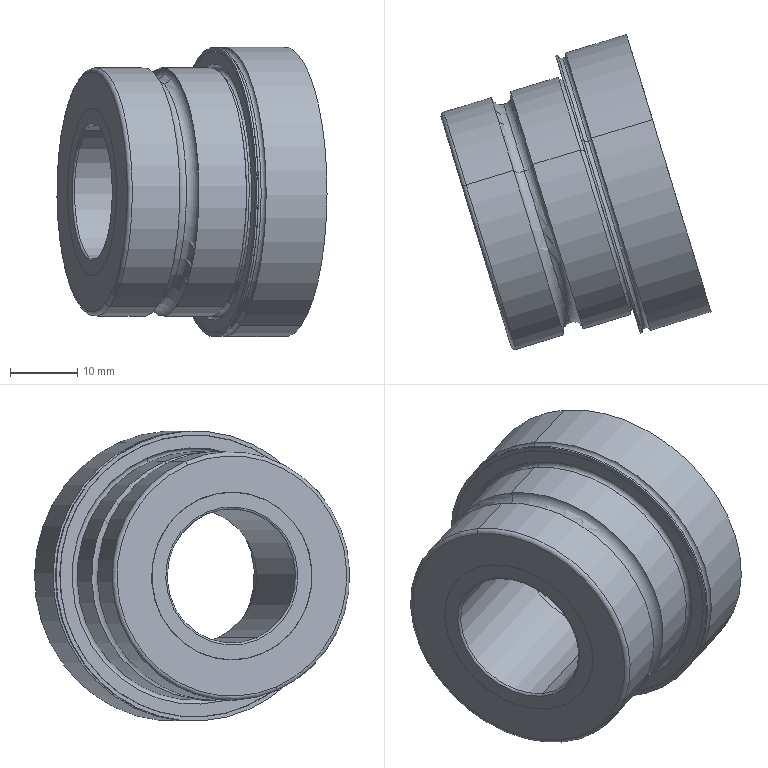Component | SolidWorks | v1ZHXTNKXRZ20SB1-1 | 1 solid | 43 faces | box 40.25 x 46.96 x 43.2 mm | volume 24773 mm3 | torus 24 | cylinder 12 | plane 7 | commonest cylinder face diameters 37 x4 43.2 x4 25 x2 20 x2
build123d program:
from build123d import *


with BuildPart() as part:
    # Sketch1 → Revolve1 (revolve)
    with BuildSketch(Plane.XY, mode=Mode.PRIVATE) as revolve1_sk:
        with BuildLine():
            Line((0, 21.6), (0, 18.87))
            ThreePointArc((0, 18.87), (0.02, 18.85), (0, 18.83))
            Line((0, 18.83), (0, 13.1))
            ThreePointArc((0, 13.1), (0.1757, 12.676), (0.6, 12.5))
            Line((0.6, 12.5), (10, 12.5))
            Line((10, 12.5), (10, 10))
            Line((10, 10), (29.7, 10))
            ThreePointArc((29.7, 10), (29.912, 10.088), (30, 10.3))
            Line((30, 10.3), (30, 12.48))
            ThreePointArc((30, 12.48), (29.98, 12.5), (30, 12.52))
            Line((30, 12.52), (30, 17.9))
            ThreePointArc((30, 17.9), (29.824, 18.324), (29.4, 18.5))
            Line((29.4, 18.5), (22, 18.5))
            ThreePointArc((22, 18.5), (20.5, 17), (19, 18.5))
            Line((19, 18.5), (11.6, 18.5))
            ThreePointArc((11.6, 18.5), (10.576, 18.076), (11, 19.1))
            Line((11, 19.1), (11, 20.98))
            ThreePointArc((11, 20.98), (10.98, 21), (11, 21.02))
            Line((11, 21.02), (11, 21.6))
            Line((11, 21.6), (10.683, 21.6))
            ThreePointArc((10.683, 21.6), (10.083, 21), (9.483, 21.6))
            Line((9.483, 21.6), (0, 21.6))
        make_face()
    revolve(revolve1_sk.sketch.rotate(Axis((30, 0, 0), (-1, 0, 0)), 270), axis=Axis((30, 0, 0), (-1, 0, 0)))


solid = part.part

# Placed as in the assembly
solid = solid.moved(Location((237.932, -213.623, 375.239), (30.764, 8.87, -165.477)))